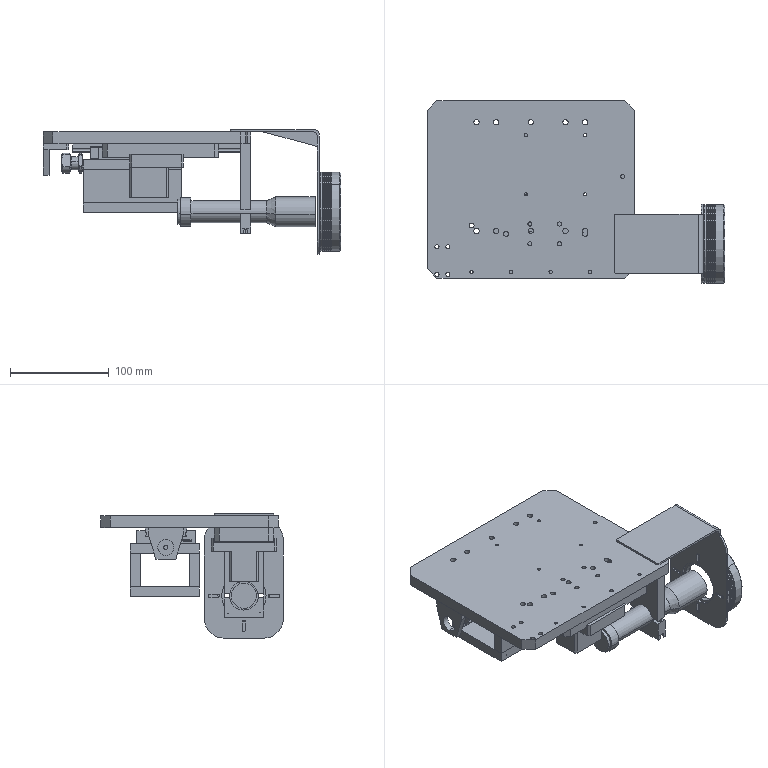Assembly | SolidWorks | mm | 15 component files | 16 solids | 956 faces | box 301.44 x 185 x 126 mm | volume 1083130 mm3 | cylinder 441 | plane 397 | cone 56 | spline 44 | sphere 14 | torus 4 | commonest cylinder face diameters 4.5 x65 4.2 x62 8 x59 3.3 x38 5.5 x37 4 x32 10 x29 5 x18
Bill of materials:
01-1111 | 1 | 1060 Alloy | Thin, nearly square flat plate with chamfered corners and many small through-holes spread across it in an irregular pattern.
05-1111 | 1 | Plain Carbon Steel | Block-shaped bracket: a rectangular top flange with four through-holes, and below it a tapered (trapezoidal) web with one large round through-bore.
06-1111 | 1 |  | Spool- or bobbin-shaped solid of revolution: two coaxial end flanges joined by a smaller-diameter cylindrical neck. Each flange is a disc with two parallel flats (double-D profile) and chamfered outer edges. One flange is axially much thicker than the other. A small central axial hole runs along the axis and appears to pass all the way through.
07-1111 | 2 | AL6061(GB)Natural Anodized | Plain rectangular bar/block with two small through-holes on its narrow top face, spaced along its length.
08-1111 | 2 | AL6061 | Rectangular flat plate with sharp corners and eight through-holes: three along each long edge and two more on the center line.
09-1111 | 1 | AL6061(GB)Natural Anodized | Upright rectangular plate/block with a semicircular cutout centered on its bottom edge and two holes in its narrow top face.
10-1111 | 1 | AL6061(GB)Natural Anodized | Rectangular block with a large semicircular saddle cut into its top, a vertical through-hole on each side of the saddle, and small slots/notches at the bottom.
123456789-DL-OP20-ST12--002-1111 | 1 | AL6061 Hard Anodized Surface | Rectangular thick plate with chamfered corners, two edge rows of eight small holes each, and six larger holes in the middle area.
123456789-DL-OP20-ST12--003-1111 | 1 | AL6061 Surface Hard Anodized | T-section block: a wide top plate with raised lips along two opposite edges, four long slots and three countersunk/counterbored holes, sitting on a narrower rectangular boss below.
123456789-DL-OP20-ST12--004-1111 | 1 | AL6061 | Thin bent sheet-like L-bracket: a flat rectangular leg plus a perpendicular leg with rounded corners that has a large central round hole surrounded by four radial slots.
C1509014-VR80-60-B-A-1111 | 1 |  | Short, thick-walled ring with several shallow circumferential grooves on its outer surface, an inward lip at one end, and four pairs of small pegs on the inner face of the lip.
Lens-1111 | 1 |  | Stepped round pin/shaft: a short collar near one end with a small end spigot, a long slimmer middle section, and a tapered step up to a larger-diameter solid cylinder at the other end.
MGW15H-1111 | 1 |  | Long rectangular plate/rail with two rows of through-holes and a long line along its center, combined with a shorter, wider block section underneath that sticks out on both sides.
Mates:
1. coincident | 01-1111-1 plane at (0, 0, 0) dir (0, 0, 1) | assembly plane at (0, 0, 0) dir (0, 0, 1)
2. coincident | 01-1111-1 plane at (0, 0, 0) dir (0, 1, 0) | assembly plane at (0, 0, 0) dir (0, 1, 0)
3. coincident | 01-1111-1 plane at (0, 0, 0) dir (1, 0, 0) | assembly plane at (0, 0, 0) dir (1, 0, 0)
4. parallel | 01-1111-1 face at (0, 0, -6) dir (0, 0, -1) | ImagingSystem-1111-1/123456789-DL-OP20-ST12--002-1111-1 face at (-45, -85, -6) dir (0, 0, 1)
5. coincident | 01-1111-1 face at (0, 0, -6) dir (0, 0, -1) | MGW15H-1111-1 face at (-75, 3, -6) dir (0, 0, 1)
6. parallel | 01-1111-1 face at (-105, -90, 6) dir (0, -1, 0) | MGW15H-1111-1 face at (-56.9, -6, -9.4) dir (0, -1, 0)
7. coincident | 01-1111-1 face at (105, 90, 6) dir (1, 0, 0) | MGW15H-1111-1 face at (105, 3, -12.4) dir (1, 0, 0)
8. coincident | 01-1111-1 face at (0, 0, -6) dir (0, 0, -1) | 05-1111-1 face at (-79, 6, -6) dir (0, 0, 1)
9. parallel | 01-1111-1 face at (-105, 90, 6) dir (-1, 0, 0) | 05-1111-1 face at (-105, 6, -6) dir (-1, 0, 0)
10. coincident | 01-1111-1 face at (-105, 90, 6) dir (-1, 0, 0) | 05-1111-1 face at (-105, 6, -6) dir (-1, 0, 0)
11. coincident | 01-1111-1 face at (0, 0, -6) dir (0, 0, -1) | ImagingSystem-1111-1/123456789-DL-OP20-ST12--002-1111-1 face at (-45, -85, -6) dir (0, 0, 1)
12. coincident | 07-1111-1 face at (-64.57, 60, -66) dir (-1, 0, 0) | 07-1111-2 face at (-64.57, 0, -66) dir (-1, 0, 0)
13. coincident | 07-1111-1 face at (-64.57, 50, -66) dir (0, 0, -1) | 08-1111-1 face at (-64.57, 60, -66) dir (0, 0, 1)
14. coincident | 07-1111-1 face at (-64.57, 60, -66) dir (-1, 0, 0) | 08-1111-1 face at (-64.57, 60, -66) dir (-1, 0, 0)
15. coincident | 07-1111-1 face at (-64.57, 60, -66) dir (0, 1, 0) | 08-1111-1 face at (-64.57, 60, -76) dir (0, 1, 0)
16. coincident | 01-1111-1 face at (0, 0, -6) dir (0, 0, -1) | 09-1111-1 face at (95, -35, -6) dir (0, 0, 1)
17. parallel | ImagingSystem-1111-1/123456789-DL-OP20-ST12--002-1111-1 face at (73, 8.898, -6) dir (1, 0, 0) | 09-1111-1 face at (95, -35, -73) dir (-1, 0, 0)
18. width | 09-1111-1 face at (105, -35, -73) dir (0, 1, 0) | 09-1111-1 face at (105, -75, -73) dir (0, -1, 0) | assembly face at (61.294, -10, -75) dir (-1, 0, 0) r 11
19. concentric | assembly face at (61.294, -10, -75) dir (-1, 0, 0) r 11 | 10-1111-1 face at (95, -55, -75) dir (1, 0, 0) r 11
20. coincident | 09-1111-1 face at (105, -35, -73) dir (1, 0, 0) | 10-1111-1 face at (105, -75.022, -76.768) dir (1, 0, 0)
21. distance | ImagingSystem-1111-1/123456789-DL-OP20-ST12--002-1111-1 face at (-45, -85, -20) dir (-1, 0, 0) | 01-1111-1 face at (-105, 90, 6) dir (-1, 0, 0)
22. coincident | 01-1111-1 face at (105, 90, 6) dir (1, 0, 0) | 09-1111-1 face at (105, -35, -73) dir (1, 0, 0)
23. distance | MGW15H-1111-1 face at (-75, 45, -6) dir (0, 1, 0) | 01-1111-1 face at (-105, 90, 6) dir (0, 1, 0)
24. width | MGW15H-1111-1 face at (-56.9, 53.6, -9.4) dir (0, 1, 0) | MGW15H-1111-1 face at (-56.9, -5.6, -9.4) dir (0, -1, 0) | 05-1111-1 face at (-105, 42, -6) dir (0, 1, 0) | 05-1111-1 face at (-105, 6, -6) dir (0, -1, 0)
25. coincident | 07-1111-2 face at (-64.57, -10, -66) dir (0, 0, -1) | 08-1111-1 face at (-64.57, 60, -66) dir (0, 0, 1)
26. coincident | 08-1111-1 face at (-64.57, 60, -76) dir (0, 1, 0) | 08-1111-2 face at (-64.57, 60, -32) dir (0, 1, 0)
27. coincident | 07-1111-1 face at (-64.57, 50, -32) dir (0, 0, 1) | 08-1111-2 face at (-64.57, 60, -32) dir (0, 0, -1)
28. coincident | 08-1111-1 face at (-64.57, 60, -66) dir (-1, 0, 0) | 08-1111-2 face at (-64.57, 60, -22) dir (-1, 0, 0)
29. coincident | MGW15H-1111-1 face at (-56.9, -6, -22) dir (0, 0, -1) | 08-1111-2 face at (-64.57, 60, -22) dir (0, 0, 1)
30. concentric | ImagingSystem-1111-1/Lens-1111-2 face at (121.294, -55, -75) dir (-1, 0, 0) r 11 | 09-1111-1 face at (95, -55, -75) dir (1, 0, 0) r 11
31. concentric | ImagingSystem-1111-1/Lens-1111-2 face at (121.294, -55, -75) dir (-1, 0, 0) r 11 | 10-1111-1 face at (95, -55, -75) dir (1, 0, 0) r 11
32. distance | ImagingSystem-1111-1/123456789-DL-OP20-ST12--002-1111-1 face at (-45, -85, -6) dir (0, -1, 0) | 01-1111-1 face at (-105, -90, 6) dir (0, -1, 0)
33. coincident | 123456789-DL-OP20-ST12--002-1111-1 face at (36.704, -40.189, -257.423) dir (0, -1, 0) | 123456789-DL-OP20-ST12--003-1111-1 face at (84.111, -40.189, -185.282) dir (0, 1, 0)
34. coincident | 123456789-DL-OP20-ST12--002-1111-1 face at (96.704, -26.189, -257.423) dir (1, 0, 0) | 123456789-DL-OP20-ST12--003-1111-1 face at (96.704, -37.189, -175.739) dir (-1, 0, 0)
35. concentric | C1509014-VR80-60-B-A-1111-1 face at (66.704, -95.189, 38.438) dir (0, 0, 1) r 20 | 123456789-DL-OP20-ST12--004-1111-1 face at (66.704, -95.189, -47.982) dir (0, 0, -1) r 22.5
36. coincident | 123456789-DL-OP20-ST12--004-1111-1 face at (106.704, -138.189, -37.982) dir (0, 0, 1) | C1509014-VR80-60-B-A-1111-1 face at (52.777, -109.543, -37.982) dir (0, 0, -1)
37. width | 123456789-DL-OP20-ST12--004-1111-1 face at (96.704, -138.189, -42.982) dir (1, 0, 0) | 123456789-DL-OP20-ST12--004-1111-1 face at (36.704, -138.189, -42.982) dir (-1, 0, 0) | 123456789-DL-OP20-ST12--002-1111-1 face at (96.704, -26.189, -257.423) dir (1, 0, 0) | 123456789-DL-OP20-ST12--002-1111-1 face at (36.704, -26.189, -257.423) dir (-1, 0, 0)